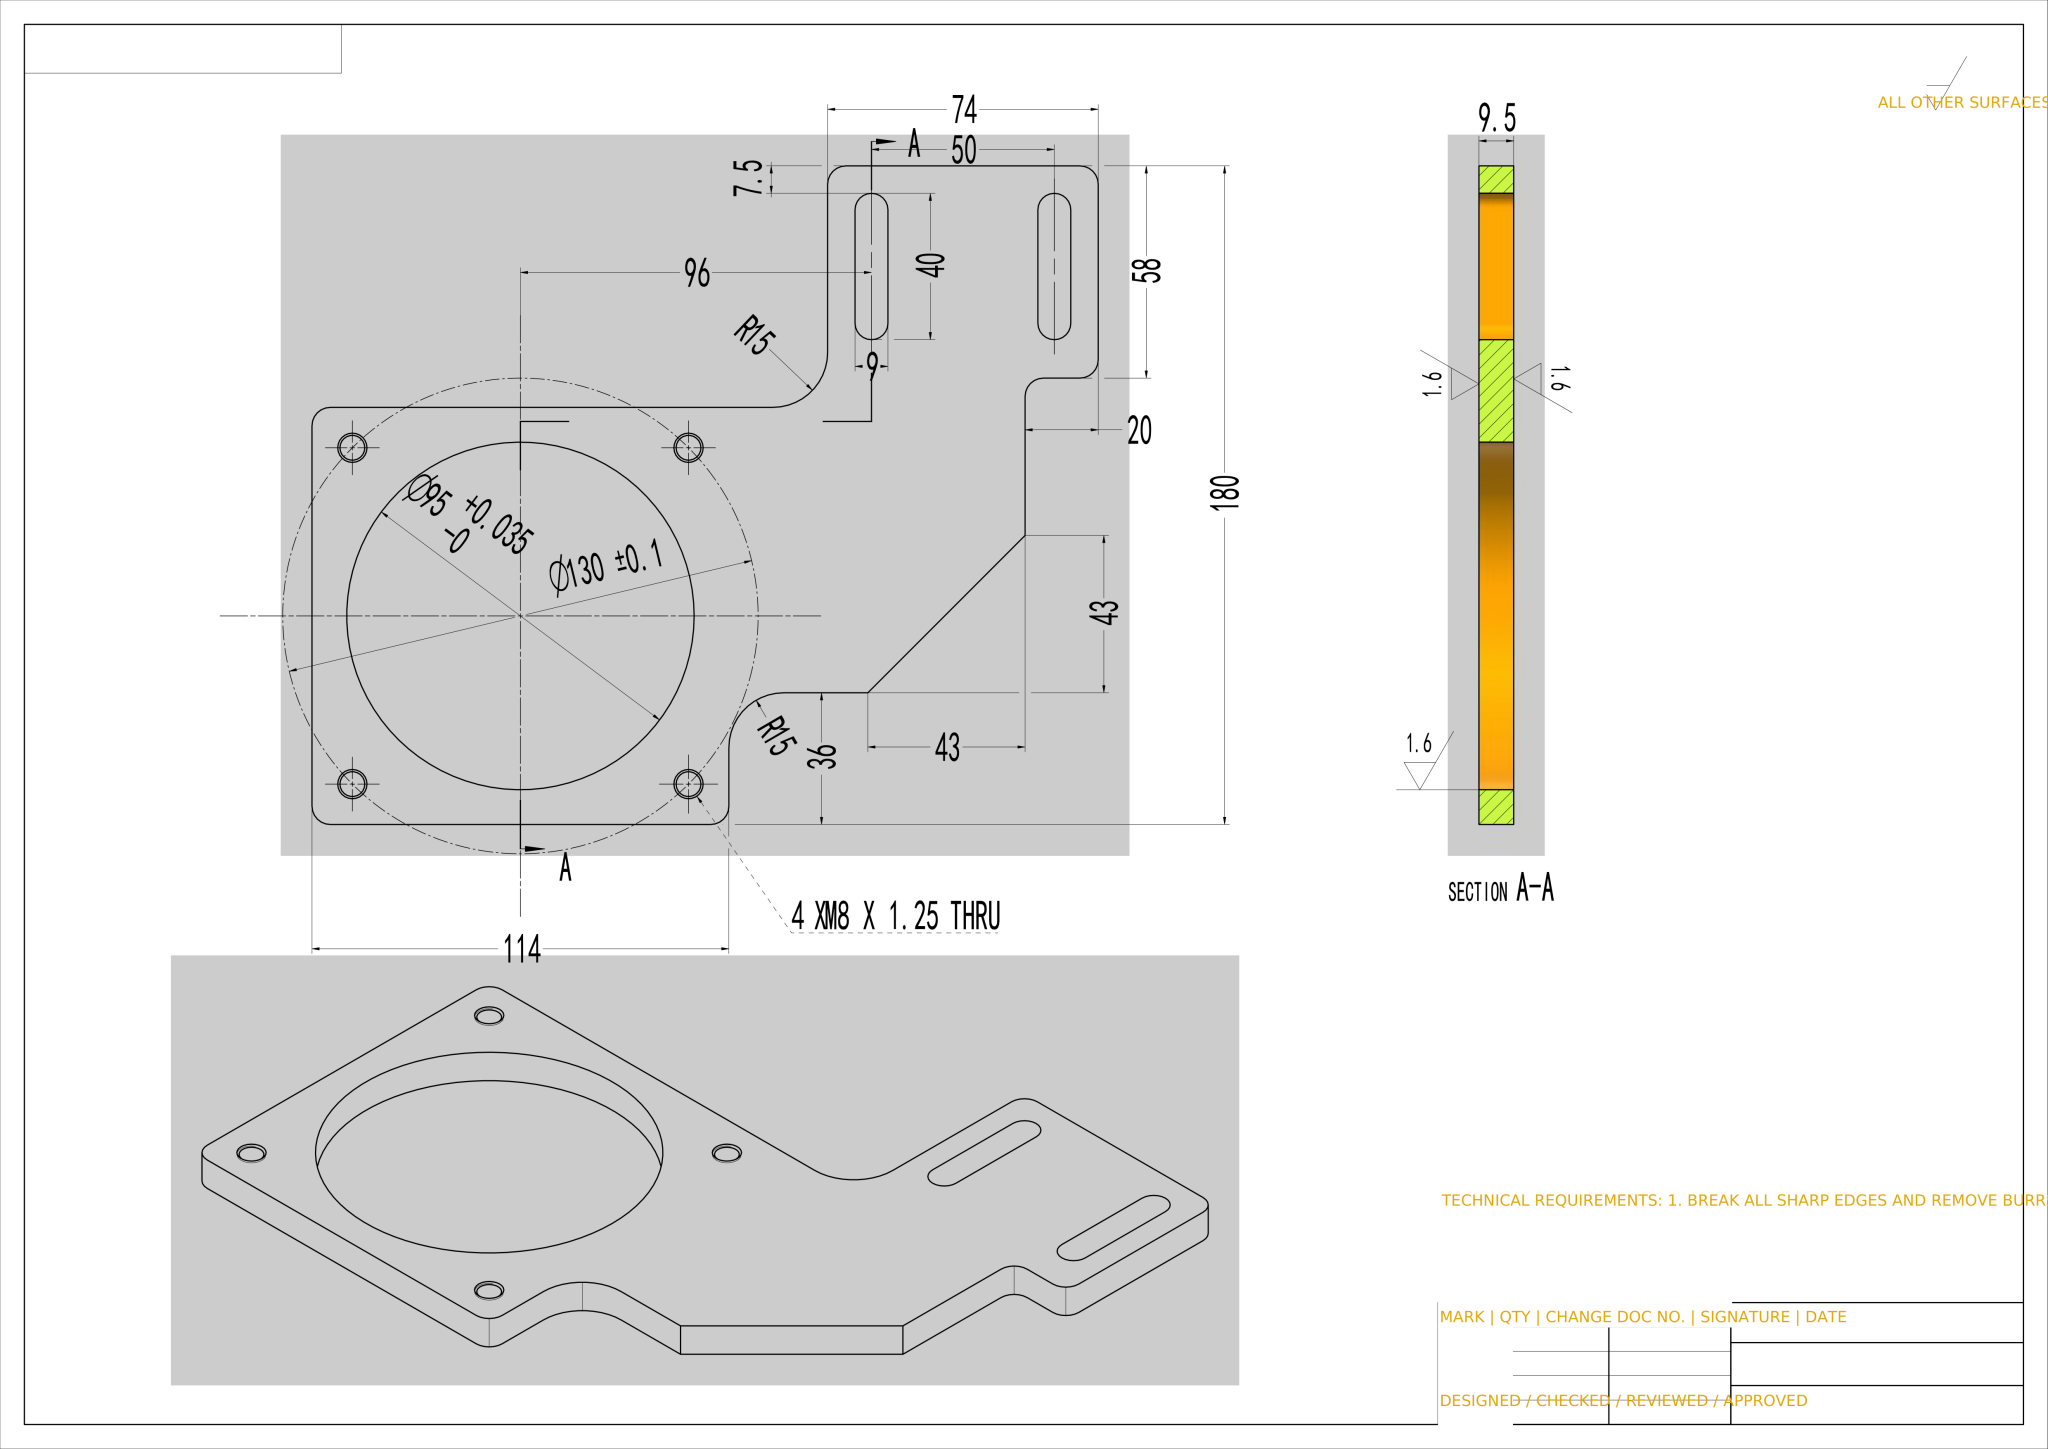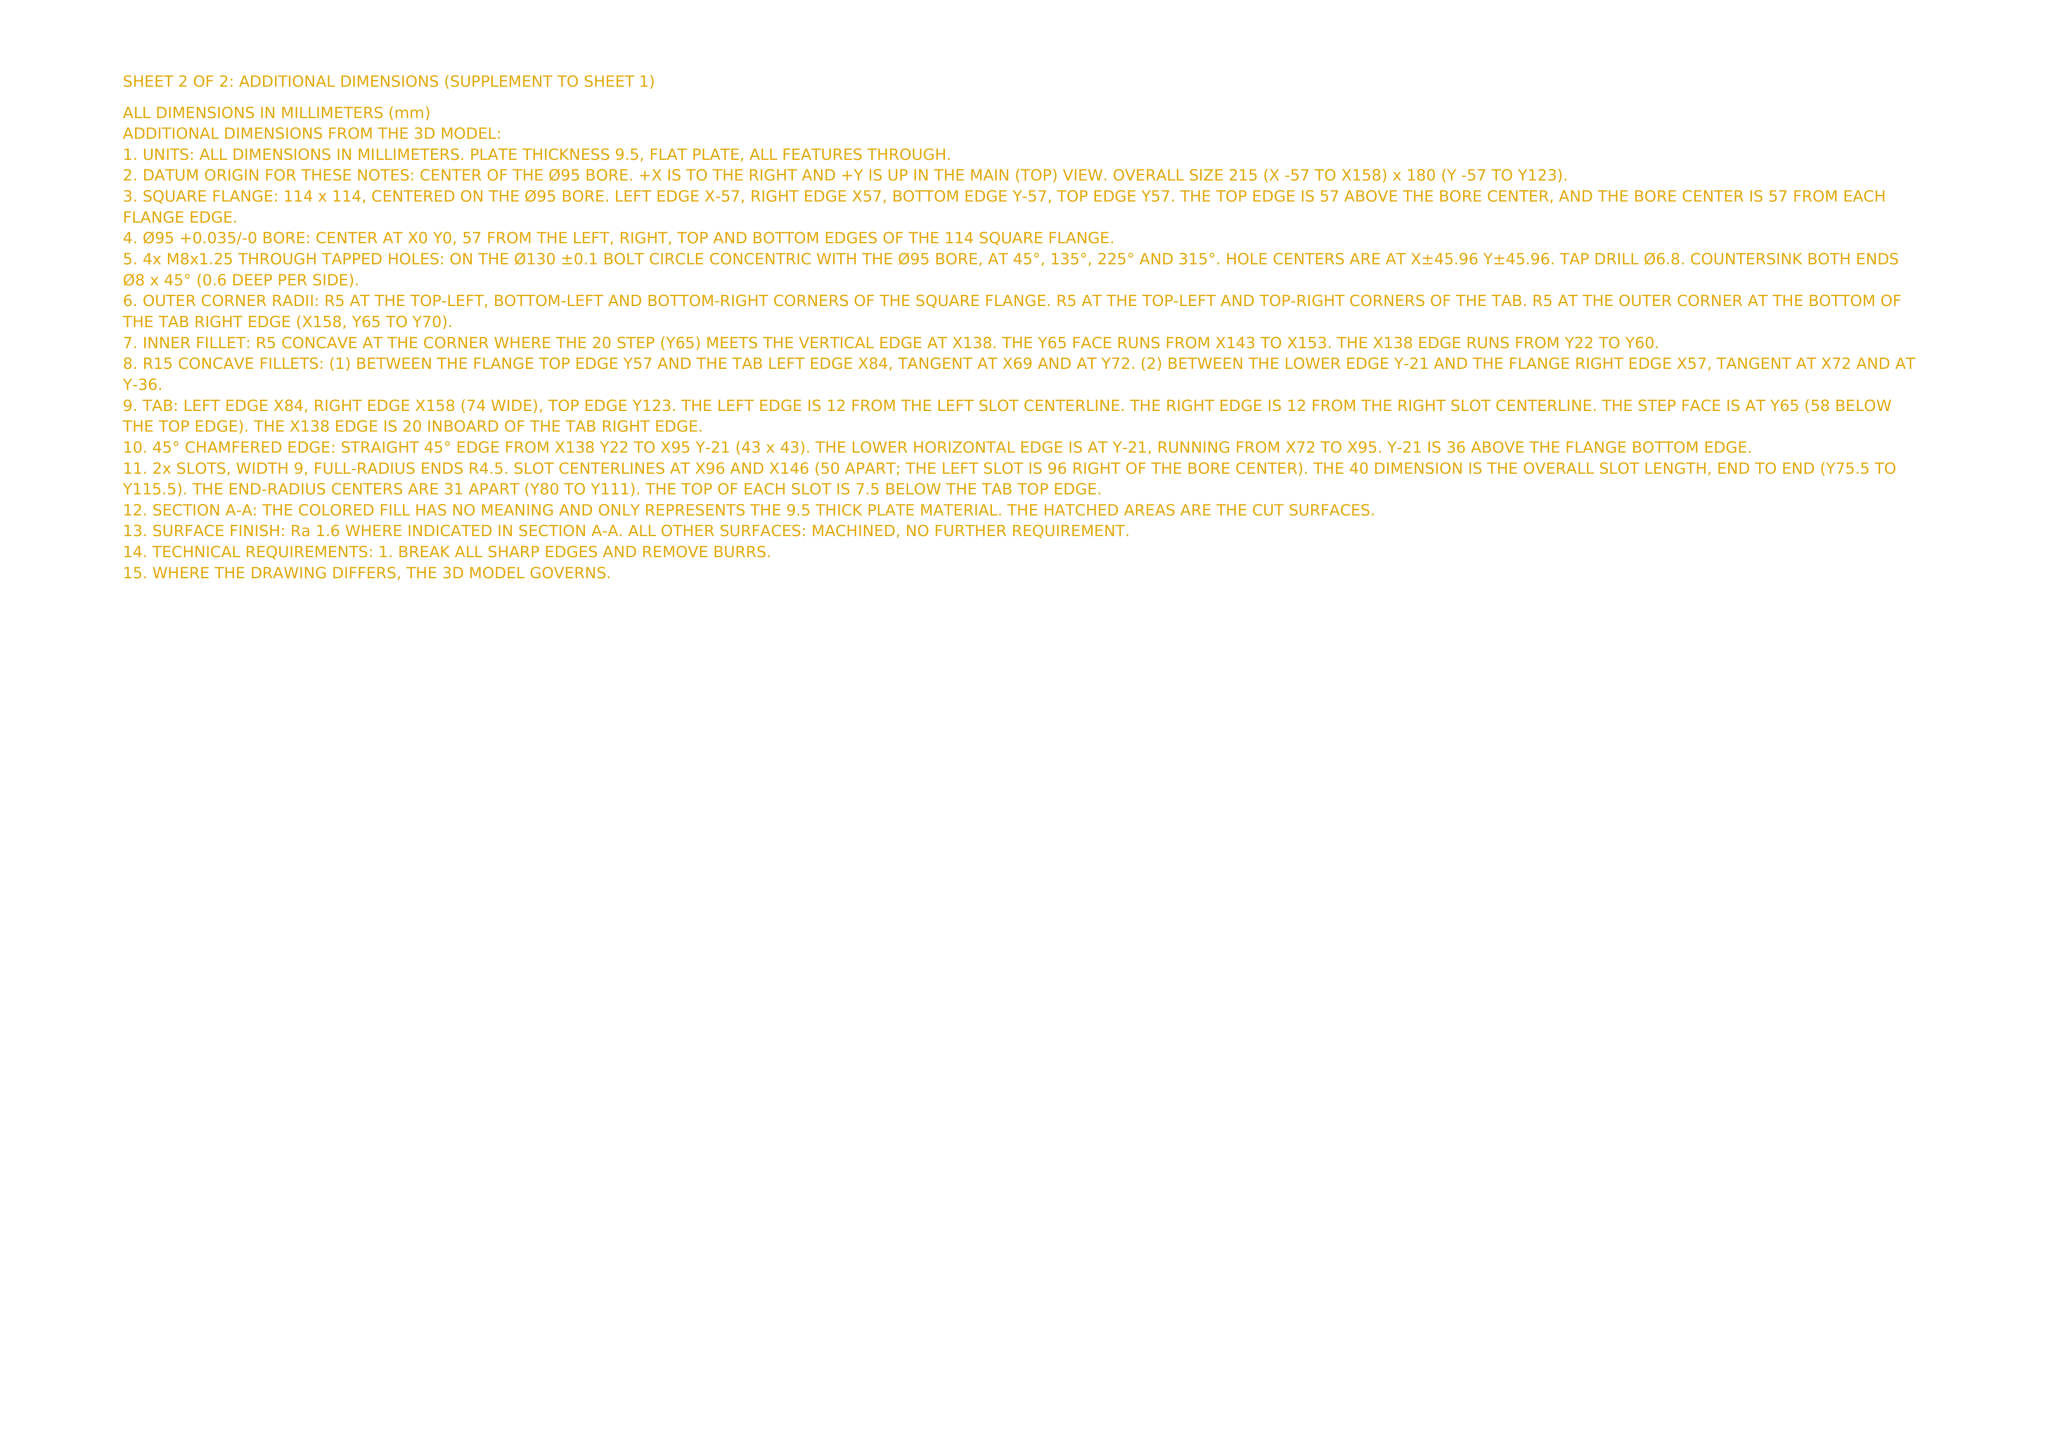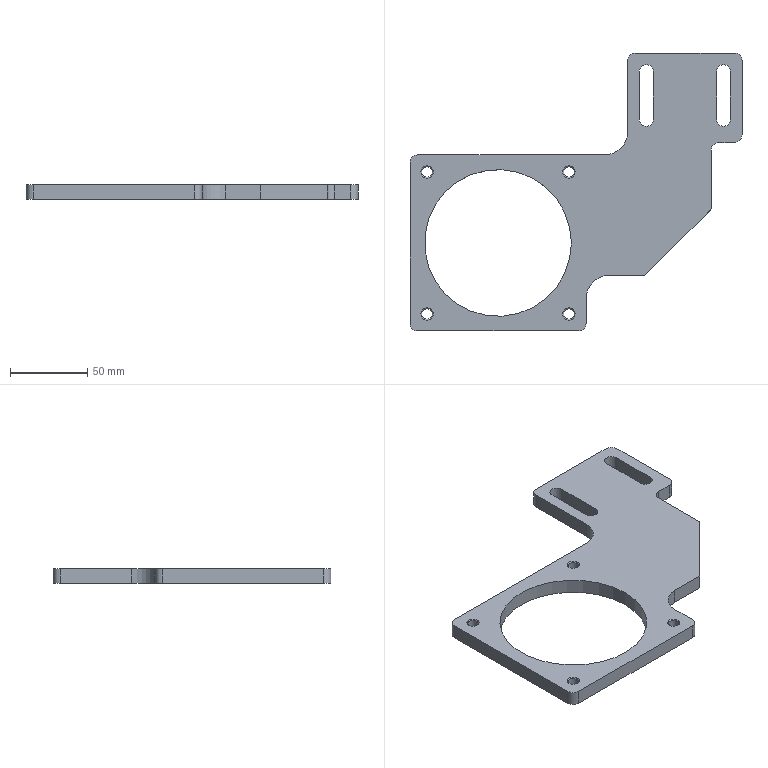Part | NX | mm | 1 solid | 43 faces | box 215 x 180 x 9.5 mm | volume 144980 mm3 | cylinder 18 | plane 17 | cone 8 | commonest cylinder face diameters 10 x7 9 x4 6.8 x4 30 x2 95 x1